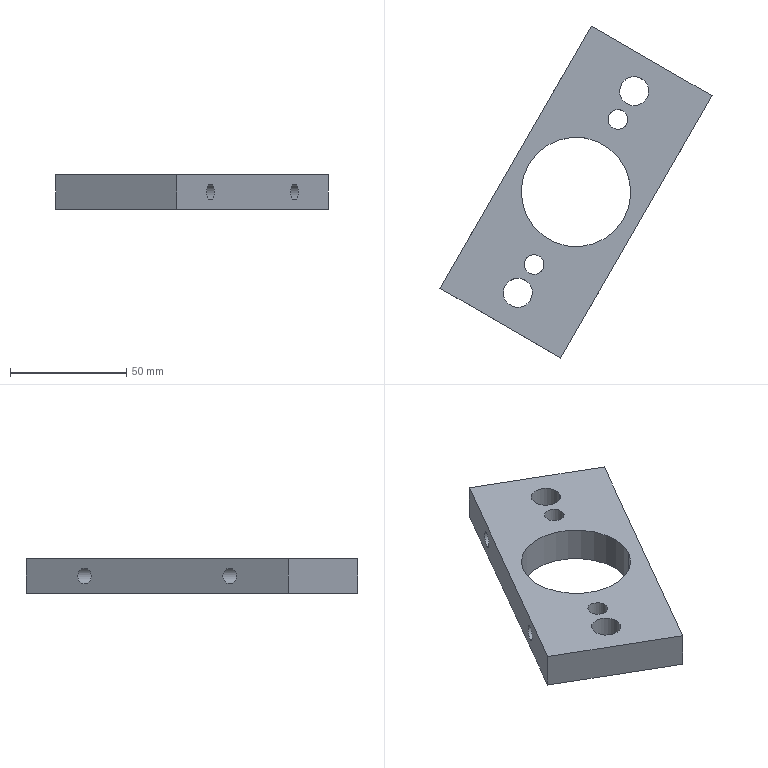Component | SolidWorks | SpindleFixtureAssemblyLeft-1_KLHFH015_38LocatingPinLimitPlate-1 | 1 solid | 24 faces | box 116.96 x 142.58 x 15 mm | volume 81797 mm3 | cylinder 18 | plane 6 | commonest cylinder face diameters 6.8 x8 8.5 x4 12.5 x4 47 x2 | material Plain Carbon Steel
build123d program:
from build123d import *

# Parameters (mm, degrees)
SKETCH1_W           = 60
SKETCH1_H           = 130
BOSS_EXTRUDE1_DEPTH = 7.5
SKETCH2_R           = 23.5
CUT_EXTRUDE1_DEPTH  = 74.144
SKETCH5_R           = 6.25
CUT_EXTRUDE2_DEPTH  = 74.144
M10_TAPPED_HOLE1_D  = 8.5
M8_TAPPED_HOLE1_D   = 6.8


with BuildPart() as part:
    # Sketch1 → Boss-Extrude1 (new, symmetric)
    with BuildSketch(Plane.XY):
        Rectangle(SKETCH1_W, SKETCH1_H)
    extrude(amount=BOSS_EXTRUDE1_DEPTH, both=True)

    # Sketch2 → Cut-Extrude1 (cut, through all)
    with BuildSketch(Plane.XY.offset(7.5)):
        Circle(SKETCH2_R)
    extrude(amount=-CUT_EXTRUDE1_DEPTH, mode=Mode.SUBTRACT)

    # Sketch5 → Cut-Extrude2 (cut, through all)
    with BuildSketch(Plane.XY.offset(-7.5)):
        with Locations((0, 50)):
            Circle(SKETCH5_R)
        with Locations((0, -50)):
            Circle(SKETCH5_R)
    extrude(amount=CUT_EXTRUDE2_DEPTH, mode=Mode.SUBTRACT)

    # M10 Tapped Hole1 (through all)
    with Locations(Plane(origin=(0, 0, -7.5), x_dir=(-1, 0, 0), z_dir=(0, 0, -1))):
        with Locations((0, 36), (0, -36)):
            Hole(M10_TAPPED_HOLE1_D / 2)

    # M8 Tapped Hole1 (through all)
    with Locations(Plane(origin=(30, 0, 0), x_dir=(0, 0, -1), z_dir=(1, 0, 0))):
        with Locations((0, 36), (0, -36)):
            Hole(M8_TAPPED_HOLE1_D / 2)


solid = part.part

# Placed as in the assembly
solid = solid.moved(Location((0, 0, -262), (0, 0, -30)))